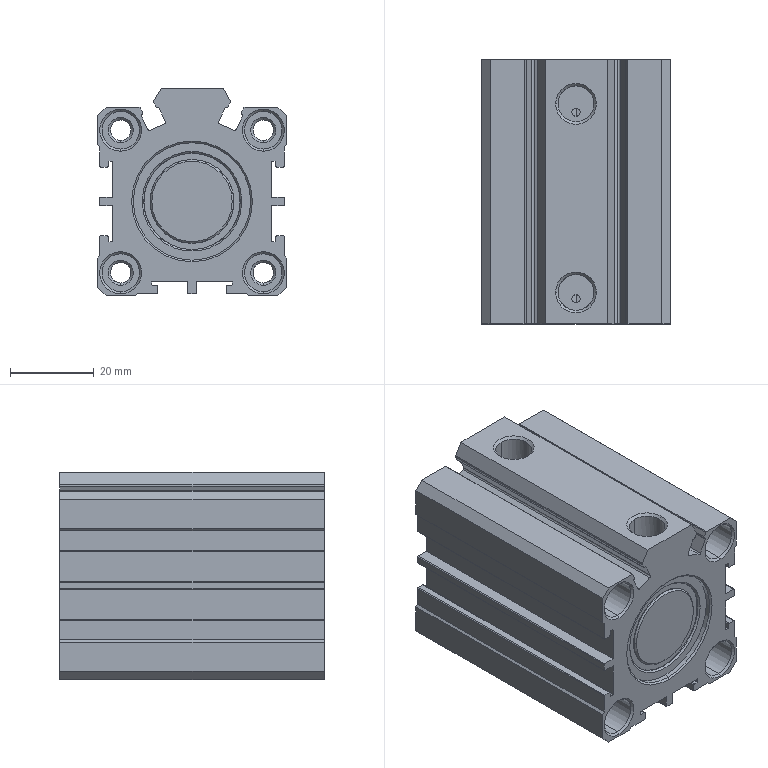Component | SolidWorks | SL021-113Q32x30S-2.SL41SM-1_SL021-113Q32x30S (2)-2.sl4prt-1 | 1 solid | 242 faces | volume 66486 mm3 | cylinder 104 | plane 92 | cone 44 | spline 2 | commonest cylinder face diameters 0.4 x36 9 x16 2 x8 4.917 x8 0.8 x8 8.566 x4 23 x4 3.8 x4